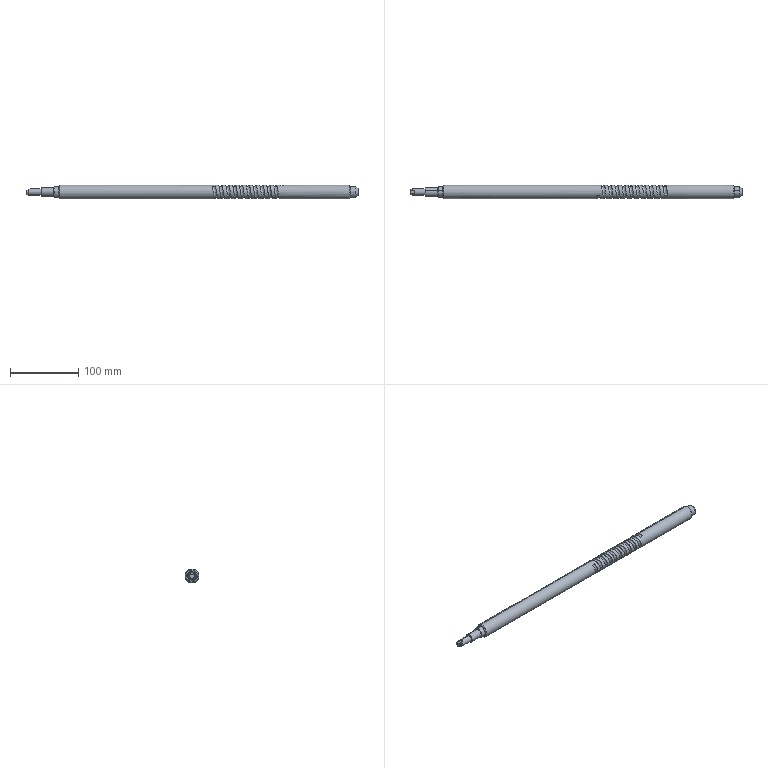Component | SolidWorks | BallScrew-1 | 1 solid | 58 faces | volume 135339 mm3 | cylinder 30 | plane 13 | cone 12 | spline 3 | commonest cylinder face diameters 20 x21 15 x4 9.527 x2 12.431 x2 7.469 x1